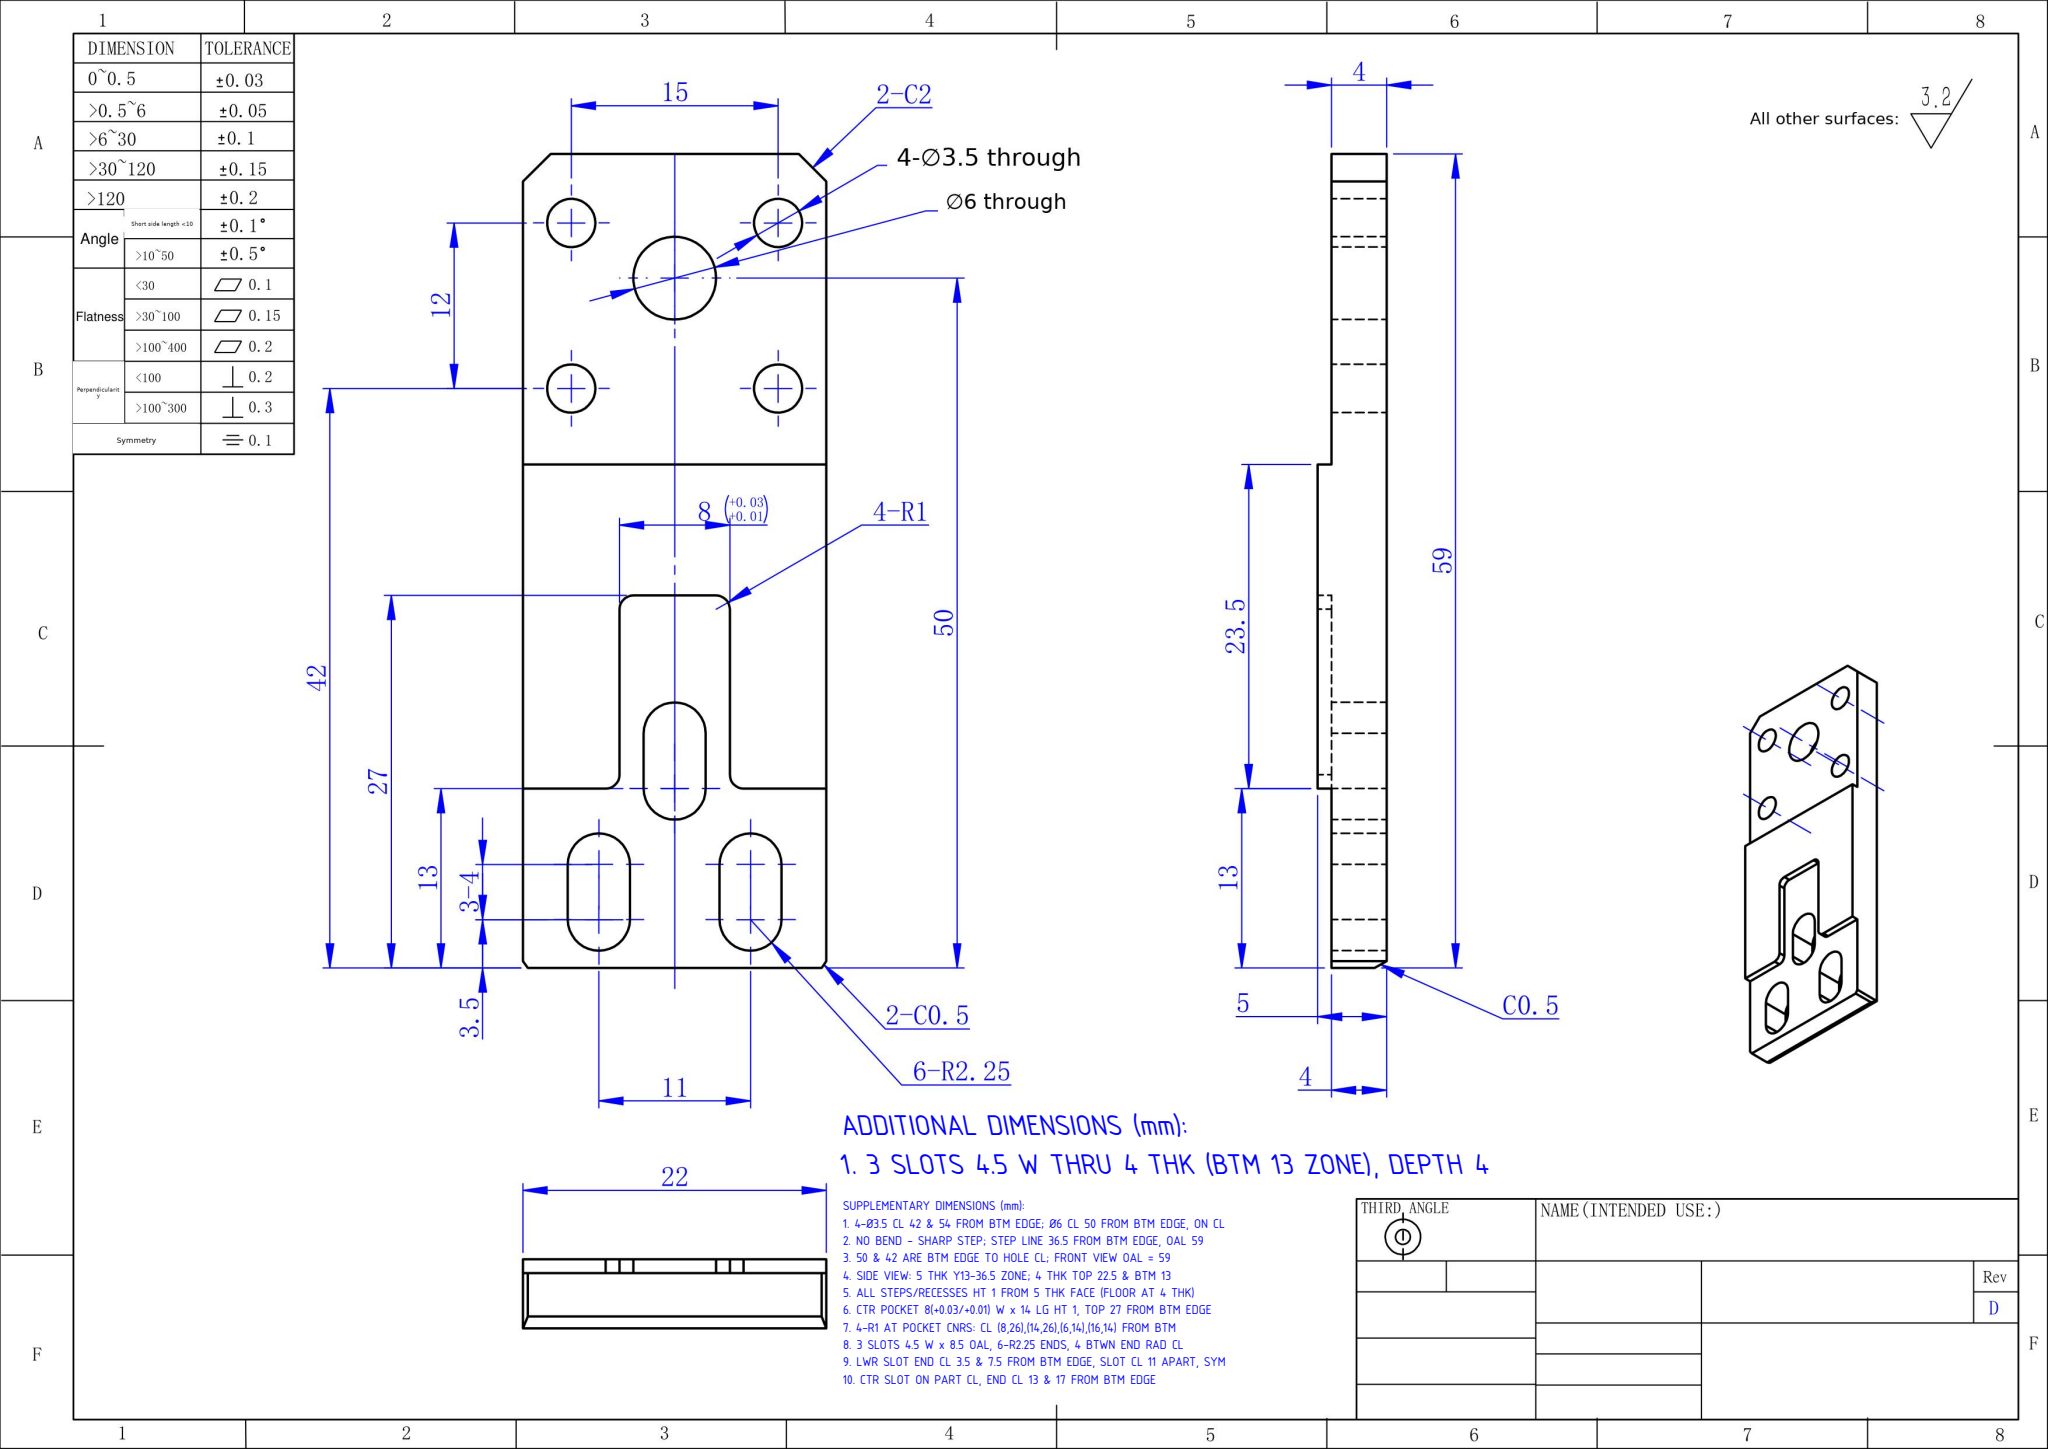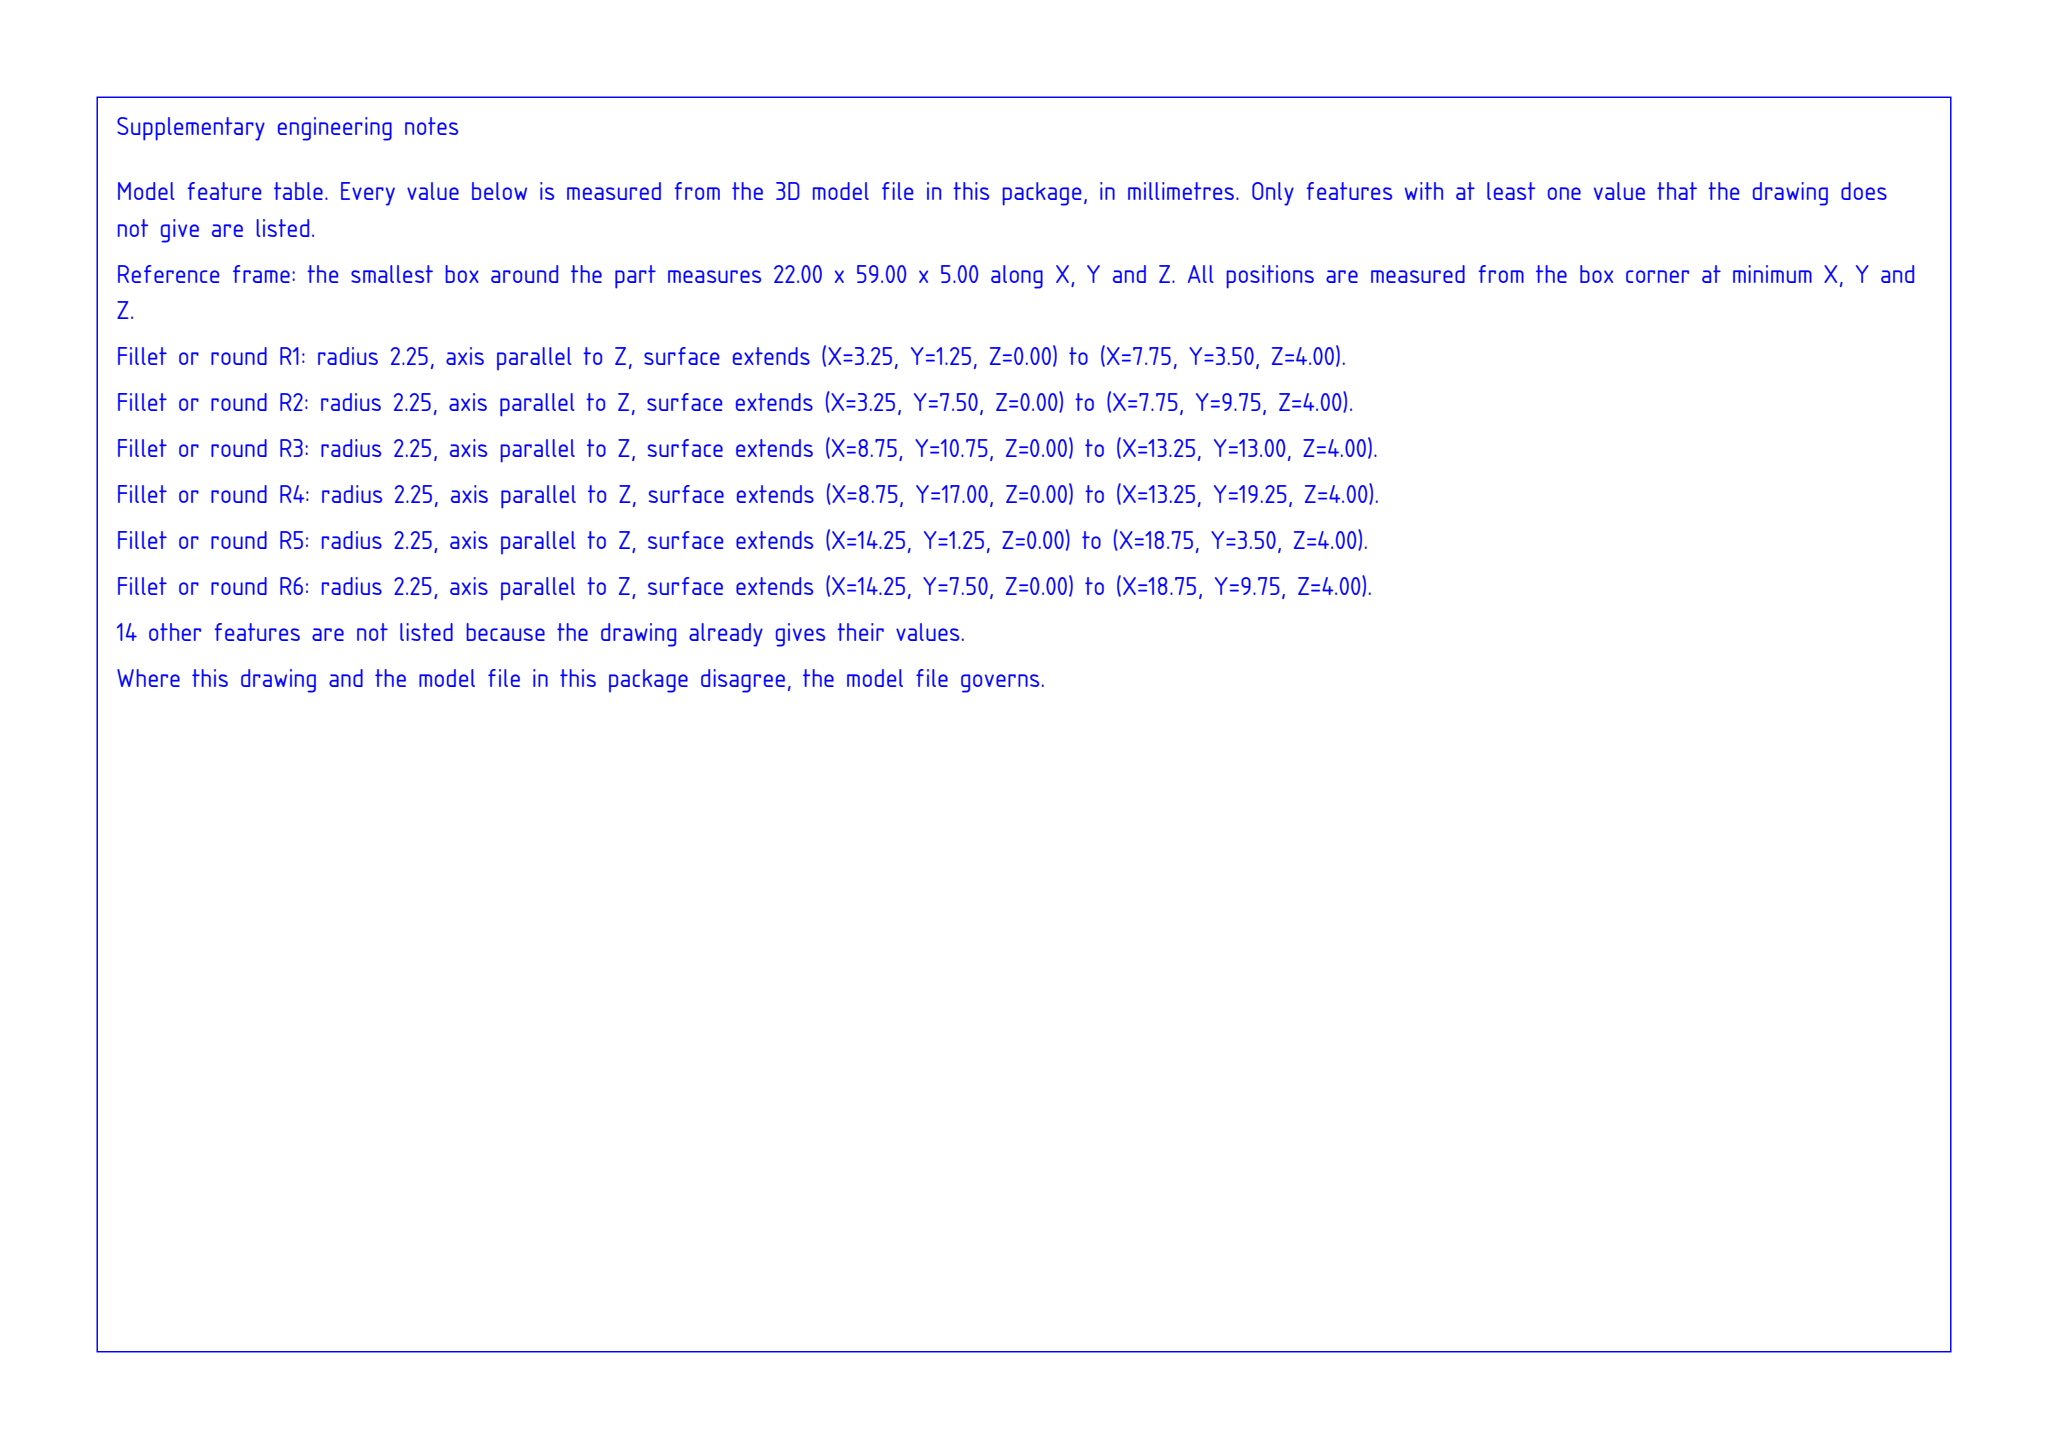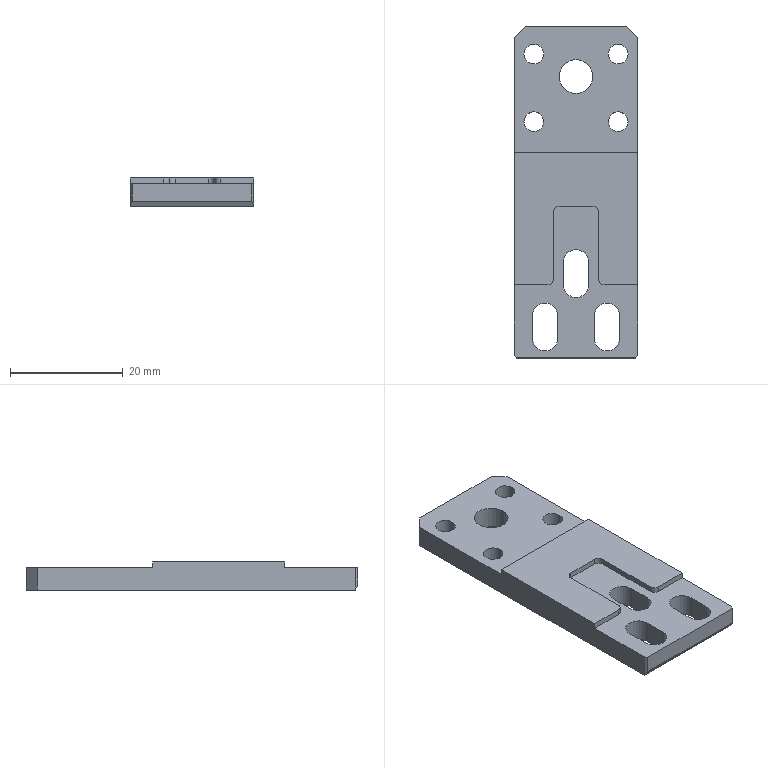Part | SolidWorks | mm | 1 solid | 45 faces | box 22 x 59 x 5 mm | volume 4902 mm3 | plane 25 | cylinder 20 | commonest cylinder face diameters 3.5 x8 4.5 x6 2 x4 6 x2